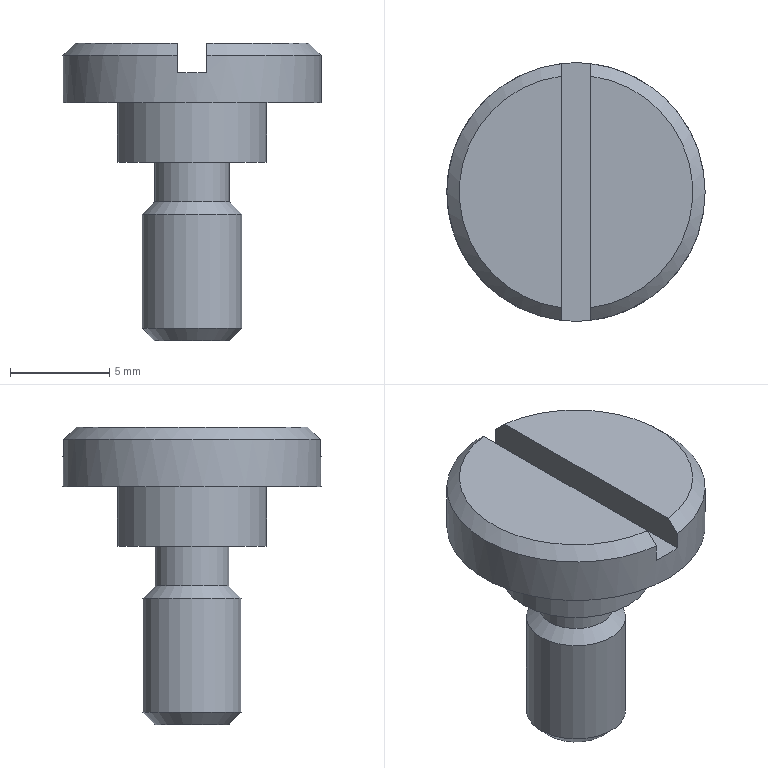Component | NX | DRILL_BUSHING_SCREW | 1 solid | 16 faces | box 13.01 x 13.01 x 15 mm | volume 650 mm3 | plane 8 | cone 4 | cylinder 4 | commonest cylinder face diameters 13.012 x1 7.512 x1 3.748 x1 5 x1
STEP:
#1=CARTESIAN_POINT('',(0.,0.,0.));
#2=DIRECTION('',(0.,0.,1.));
#3=DIRECTION('',(1.,0.,0.));
#4=AXIS2_PLACEMENT_3D('',#1,#2,#3);
#5=CARTESIAN_POINT('',(-1.25,94.806,-197.498));
#6=VERTEX_POINT('',#5);
#7=CARTESIAN_POINT('',(-1.25,106.47,-197.498));
#8=VERTEX_POINT('',#7);
#9=CARTESIAN_POINT('',(-1.25,86.638,-197.498));
#10=DIRECTION('',(0.,1.,0.));
#11=VECTOR('',#10,1.);
#12=LINE('',#9,#11);
#13=CARTESIAN_POINT('',(-2.,100.638,-197.498));
#14=DIRECTION('',(0.,0.,1.));
#15=DIRECTION('',(1.,0.,-0.));
#16=AXIS2_PLACEMENT_3D('',#13,#14,#15);
#17=PLANE('',#16);
#18=CARTESIAN_POINT('',(0.75,-14.));
#19=DIRECTION('',(0.,1.));
#20=VECTOR('',#19,1.);
#21=LINE('',#18,#20);
#22=(GEOMETRIC_REPRESENTATION_CONTEXT(2)PARAMETRIC_REPRESENTATION_CONTEXT()REPRESENTATION_CONTEXT('',''));
#23=DEFINITIONAL_REPRESENTATION('',(#21),#22);
#24=PCURVE('',#17,#23);
#25=CARTESIAN_POINT('',(-1.25,86.638,-198.998));
#26=DIRECTION('',(1.,0.,0.));
#27=DIRECTION('',(0.,0.,-1.));
#28=AXIS2_PLACEMENT_3D('',#25,#26,#27);
#29=PLANE('',#28);
#30=CARTESIAN_POINT('',(-1.5,0.));
#31=DIRECTION('',(0.,1.));
#32=VECTOR('',#31,1.);
#33=LINE('',#30,#32);
#34=(GEOMETRIC_REPRESENTATION_CONTEXT(2)PARAMETRIC_REPRESENTATION_CONTEXT()REPRESENTATION_CONTEXT('',''));
#35=DEFINITIONAL_REPRESENTATION('',(#33),#34);
#36=PCURVE('',#29,#35);
#37=SURFACE_CURVE('',#12,(#24,#36),.PCURVE_S1.);
#38=EDGE_CURVE('',#6,#8,#37,.T.);
#39=ORIENTED_EDGE('',*,*,#38,.F.);
#40=CARTESIAN_POINT('',(-2.,100.638,-197.498));
#41=DIRECTION('',(0.,0.,1.));
#42=DIRECTION('',(1.,0.,-0.));
#43=AXIS2_PLACEMENT_3D('',#40,#41,#42);
#44=CIRCLE('',#43,5.88);
#45=CARTESIAN_POINT('',(0.,0.));
#46=DIRECTION('',(1.,0.));
#47=AXIS2_PLACEMENT_2D('',#45,#46);
#48=CIRCLE('',#47,5.88);
#49=(GEOMETRIC_REPRESENTATION_CONTEXT(2)PARAMETRIC_REPRESENTATION_CONTEXT()REPRESENTATION_CONTEXT('',''));
#50=DEFINITIONAL_REPRESENTATION('',(#48),#49);
#51=PCURVE('',#17,#50);
#52=CARTESIAN_POINT('',(-2.,100.638,-198.12));
#53=DIRECTION('',(-0.,0.,-1.));
#54=DIRECTION('',(-1.,0.,0.));
#55=AXIS2_PLACEMENT_3D('',#52,#53,#54);
#56=CONICAL_SURFACE('',#55,6.506,0.7886);
#57=CARTESIAN_POINT('',(9.425,-0.622));
#58=DIRECTION('',(-1.,0.));
#59=VECTOR('',#58,1.);
#60=LINE('',#57,#59);
#61=(GEOMETRIC_REPRESENTATION_CONTEXT(2)PARAMETRIC_REPRESENTATION_CONTEXT()REPRESENTATION_CONTEXT('',''));
#62=DEFINITIONAL_REPRESENTATION('',(#60),#61);
#63=PCURVE('',#56,#62);
#64=SURFACE_CURVE('',#44,(#51,#63),.PCURVE_S1.);
#65=EDGE_CURVE('',#6,#8,#64,.T.);
#66=ORIENTED_EDGE('',*,*,#65,.T.);
#67=EDGE_LOOP('',(#39,#66));
#68=FACE_BOUND('',#67,.T.);
#69=ADVANCED_FACE('',(#68),#17,.T.);
#70=CARTESIAN_POINT('',(-1.25,94.176,-198.12));
#71=VERTEX_POINT('',#70);
#72=CARTESIAN_POINT('',(4.506,100.638,-198.12));
#73=VERTEX_POINT('',#72);
#74=CARTESIAN_POINT('',(-2.,100.638,-198.12));
#75=DIRECTION('',(0.,0.,1.));
#76=DIRECTION('',(1.,0.,-0.));
#77=AXIS2_PLACEMENT_3D('',#74,#75,#76);
#78=CIRCLE('',#77,6.506);
#79=CARTESIAN_POINT('',(9.425,-0.));
#80=DIRECTION('',(-1.,0.));
#81=VECTOR('',#80,1.);
#82=LINE('',#79,#81);
#83=(GEOMETRIC_REPRESENTATION_CONTEXT(2)PARAMETRIC_REPRESENTATION_CONTEXT()REPRESENTATION_CONTEXT('',''));
#84=DEFINITIONAL_REPRESENTATION('',(#82),#83);
#85=PCURVE('',#56,#84);
#86=CARTESIAN_POINT('',(-2.,100.638,-192.998));
#87=DIRECTION('',(0.,0.,1.));
#88=DIRECTION('',(1.,0.,-0.));
#89=AXIS2_PLACEMENT_3D('',#86,#87,#88);
#90=CYLINDRICAL_SURFACE('',#89,6.506);
#91=CARTESIAN_POINT('',(0.,-5.122));
#92=DIRECTION('',(1.,0.));
#93=VECTOR('',#92,1.);
#94=LINE('',#91,#93);
#95=(GEOMETRIC_REPRESENTATION_CONTEXT(2)PARAMETRIC_REPRESENTATION_CONTEXT()REPRESENTATION_CONTEXT('',''));
#96=DEFINITIONAL_REPRESENTATION('',(#94),#95);
#97=PCURVE('',#90,#96);
#98=SURFACE_CURVE('',#78,(#85,#97),.PCURVE_S1.);
#99=EDGE_CURVE('',#71,#73,#98,.T.);
#100=ORIENTED_EDGE('',*,*,#99,.T.);
#101=CARTESIAN_POINT('',(-1.25,107.101,-198.12));
#102=VERTEX_POINT('',#101);
#103=CARTESIAN_POINT('',(-2.,100.638,-198.12));
#104=DIRECTION('',(0.,0.,1.));
#105=DIRECTION('',(1.,0.,-0.));
#106=AXIS2_PLACEMENT_3D('',#103,#104,#105);
#107=CIRCLE('',#106,6.506);
#108=CARTESIAN_POINT('',(9.425,-0.));
#109=DIRECTION('',(-1.,0.));
#110=VECTOR('',#109,1.);
#111=LINE('',#108,#110);
#112=(GEOMETRIC_REPRESENTATION_CONTEXT(2)PARAMETRIC_REPRESENTATION_CONTEXT()REPRESENTATION_CONTEXT('',''));
#113=DEFINITIONAL_REPRESENTATION('',(#111),#112);
#114=PCURVE('',#56,#113);
#115=CARTESIAN_POINT('',(-6.283,-5.122));
#116=DIRECTION('',(1.,0.));
#117=VECTOR('',#116,1.);
#118=LINE('',#115,#117);
#119=(GEOMETRIC_REPRESENTATION_CONTEXT(2)PARAMETRIC_REPRESENTATION_CONTEXT()REPRESENTATION_CONTEXT('',''));
#120=DEFINITIONAL_REPRESENTATION('',(#118),#119);
#121=PCURVE('',#90,#120);
#122=SURFACE_CURVE('',#107,(#114,#121),.PCURVE_S1.);
#123=EDGE_CURVE('',#73,#102,#122,.T.);
#124=ORIENTED_EDGE('',*,*,#123,.T.);
#125=CARTESIAN_POINT('',(-1.25,107.101,-198.12));
#126=CARTESIAN_POINT('',(-1.25,106.891,-197.913));
#127=CARTESIAN_POINT('',(-1.25,106.681,-197.705));
#128=CARTESIAN_POINT('',(-1.25,106.47,-197.498));
#129=B_SPLINE_CURVE_WITH_KNOTS('',3,(#125,#126,#127,#128),.UNSPECIFIED.,.F.,.F.,(4,4),(0.,1.),.PIECEWISE_BEZIER_KNOTS.);
#130=CARTESIAN_POINT('',(1.686,-0.));
#131=CARTESIAN_POINT('',(1.699,-0.622));
#132=B_SPLINE_CURVE_WITH_KNOTS('',1,(#130,#131),.UNSPECIFIED.,.F.,.F.,(2,2),(0.,1.),.PIECEWISE_BEZIER_KNOTS.);
#133=(GEOMETRIC_REPRESENTATION_CONTEXT(2)PARAMETRIC_REPRESENTATION_CONTEXT()REPRESENTATION_CONTEXT('',''));
#134=DEFINITIONAL_REPRESENTATION('',(#132),#133);
#135=PCURVE('',#56,#134);
#136=CARTESIAN_POINT('',(-0.878,20.463));
#137=CARTESIAN_POINT('',(-1.085,20.252));
#138=CARTESIAN_POINT('',(-1.293,20.042));
#139=CARTESIAN_POINT('',(-1.5,19.832));
#140=B_SPLINE_CURVE_WITH_KNOTS('',3,(#136,#137,#138,#139),.UNSPECIFIED.,.F.,.F.,(4,4),(0.,1.),.PIECEWISE_BEZIER_KNOTS.);
#141=(GEOMETRIC_REPRESENTATION_CONTEXT(2)PARAMETRIC_REPRESENTATION_CONTEXT()REPRESENTATION_CONTEXT('',''));
#142=DEFINITIONAL_REPRESENTATION('',(#140),#141);
#143=PCURVE('',#29,#142);
#144=SURFACE_CURVE('',#129,(#135,#143),.PCURVE_S1.);
#145=EDGE_CURVE('',#102,#8,#144,.T.);
#146=ORIENTED_EDGE('',*,*,#145,.T.);
#147=ORIENTED_EDGE('',*,*,#65,.F.);
#148=CARTESIAN_POINT('',(-1.25,94.806,-197.498));
#149=CARTESIAN_POINT('',(-1.25,94.596,-197.705));
#150=CARTESIAN_POINT('',(-1.25,94.386,-197.913));
#151=CARTESIAN_POINT('',(-1.25,94.176,-198.12));
#152=B_SPLINE_CURVE_WITH_KNOTS('',3,(#148,#149,#150,#151),.UNSPECIFIED.,.F.,.F.,(4,4),(0.,1.),.PIECEWISE_BEZIER_KNOTS.);
#153=CARTESIAN_POINT('',(4.584,-0.622));
#154=CARTESIAN_POINT('',(4.597,0.));
#155=B_SPLINE_CURVE_WITH_KNOTS('',1,(#153,#154),.UNSPECIFIED.,.F.,.F.,(2,2),(0.,1.),.PIECEWISE_BEZIER_KNOTS.);
#156=(GEOMETRIC_REPRESENTATION_CONTEXT(2)PARAMETRIC_REPRESENTATION_CONTEXT()REPRESENTATION_CONTEXT('',''));
#157=DEFINITIONAL_REPRESENTATION('',(#155),#156);
#158=PCURVE('',#56,#157);
#159=CARTESIAN_POINT('',(-1.5,8.168));
#160=CARTESIAN_POINT('',(-1.293,7.958));
#161=CARTESIAN_POINT('',(-1.085,7.748));
#162=CARTESIAN_POINT('',(-0.878,7.537));
#163=B_SPLINE_CURVE_WITH_KNOTS('',3,(#159,#160,#161,#162),.UNSPECIFIED.,.F.,.F.,(4,4),(0.,1.),.PIECEWISE_BEZIER_KNOTS.);
#164=(GEOMETRIC_REPRESENTATION_CONTEXT(2)PARAMETRIC_REPRESENTATION_CONTEXT()REPRESENTATION_CONTEXT('',''));
#165=DEFINITIONAL_REPRESENTATION('',(#163),#164);
#166=PCURVE('',#29,#165);
#167=SURFACE_CURVE('',#152,(#158,#166),.PCURVE_S1.);
#168=EDGE_CURVE('',#6,#71,#167,.T.);
#169=ORIENTED_EDGE('',*,*,#168,.T.);
#170=EDGE_LOOP('',(#100,#124,#146,#147,#169));
#171=FACE_BOUND('',#170,.T.);
#172=ADVANCED_FACE('',(#171),#56,.T.);
#173=CARTESIAN_POINT('',(-0.122,100.638,-212.498));
#174=VERTEX_POINT('',#173);
#175=CARTESIAN_POINT('',(-2.,100.638,-212.498));
#176=DIRECTION('',(0.,0.,1.));
#177=DIRECTION('',(1.,0.,-0.));
#178=AXIS2_PLACEMENT_3D('',#175,#176,#177);
#179=CIRCLE('',#178,1.878);
#180=CARTESIAN_POINT('',(-2.,100.638,-212.498));
#181=DIRECTION('',(0.,0.,1.));
#182=DIRECTION('',(1.,0.,-0.));
#183=AXIS2_PLACEMENT_3D('',#180,#181,#182);
#184=PLANE('',#183);
#185=CARTESIAN_POINT('',(0.,0.));
#186=DIRECTION('',(1.,0.));
#187=AXIS2_PLACEMENT_2D('',#185,#186);
#188=CIRCLE('',#187,1.878);
#189=(GEOMETRIC_REPRESENTATION_CONTEXT(2)PARAMETRIC_REPRESENTATION_CONTEXT()REPRESENTATION_CONTEXT('',''));
#190=DEFINITIONAL_REPRESENTATION('',(#188),#189);
#191=PCURVE('',#184,#190);
#192=CARTESIAN_POINT('',(-2.,100.638,-212.498));
#193=DIRECTION('',(0.,0.,1.));
#194=DIRECTION('',(1.,0.,-0.));
#195=AXIS2_PLACEMENT_3D('',#192,#193,#194);
#196=CONICAL_SURFACE('',#195,1.878,0.7822);
#197=CARTESIAN_POINT('',(0.,0.));
#198=DIRECTION('',(1.,0.));
#199=VECTOR('',#198,1.);
#200=LINE('',#197,#199);
#201=(GEOMETRIC_REPRESENTATION_CONTEXT(2)PARAMETRIC_REPRESENTATION_CONTEXT()REPRESENTATION_CONTEXT('',''));
#202=DEFINITIONAL_REPRESENTATION('',(#200),#201);
#203=PCURVE('',#196,#202);
#204=SURFACE_CURVE('',#179,(#191,#203),.PCURVE_S1.);
#205=EDGE_CURVE('',#174,#174,#204,.T.);
#206=ORIENTED_EDGE('',*,*,#205,.F.);
#207=EDGE_LOOP('',(#206));
#208=FACE_BOUND('',#207,.T.);
#209=ADVANCED_FACE('',(#208),#184,.F.);
#210=CARTESIAN_POINT('',(-2.75,106.47,-197.498));
#211=VERTEX_POINT('',#210);
#212=CARTESIAN_POINT('',(-2.75,94.806,-197.498));
#213=VERTEX_POINT('',#212);
#214=CARTESIAN_POINT('',(-2.75,114.638,-197.498));
#215=DIRECTION('',(0.,-1.,0.));
#216=VECTOR('',#215,1.);
#217=LINE('',#214,#216);
#218=CARTESIAN_POINT('',(-2.,100.638,-197.498));
#219=DIRECTION('',(0.,0.,1.));
#220=DIRECTION('',(1.,0.,-0.));
#221=AXIS2_PLACEMENT_3D('',#218,#219,#220);
#222=PLANE('',#221);
#223=CARTESIAN_POINT('',(-0.75,14.));
#224=DIRECTION('',(0.,-1.));
#225=VECTOR('',#224,1.);
#226=LINE('',#223,#225);
#227=(GEOMETRIC_REPRESENTATION_CONTEXT(2)PARAMETRIC_REPRESENTATION_CONTEXT()REPRESENTATION_CONTEXT('',''));
#228=DEFINITIONAL_REPRESENTATION('',(#226),#227);
#229=PCURVE('',#222,#228);
#230=CARTESIAN_POINT('',(-2.75,114.638,-198.998));
#231=DIRECTION('',(-1.,0.,0.));
#232=DIRECTION('',(0.,0.,1.));
#233=AXIS2_PLACEMENT_3D('',#230,#231,#232);
#234=PLANE('',#233);
#235=CARTESIAN_POINT('',(1.5,0.));
#236=DIRECTION('',(0.,-1.));
#237=VECTOR('',#236,1.);
#238=LINE('',#235,#237);
#239=(GEOMETRIC_REPRESENTATION_CONTEXT(2)PARAMETRIC_REPRESENTATION_CONTEXT()REPRESENTATION_CONTEXT('',''));
#240=DEFINITIONAL_REPRESENTATION('',(#238),#239);
#241=PCURVE('',#234,#240);
#242=SURFACE_CURVE('',#217,(#229,#241),.PCURVE_S1.);
#243=EDGE_CURVE('',#211,#213,#242,.T.);
#244=ORIENTED_EDGE('',*,*,#243,.F.);
#245=CARTESIAN_POINT('',(-2.,100.638,-197.498));
#246=DIRECTION('',(0.,0.,1.));
#247=DIRECTION('',(1.,0.,-0.));
#248=AXIS2_PLACEMENT_3D('',#245,#246,#247);
#249=CIRCLE('',#248,5.88);
#250=CARTESIAN_POINT('',(0.,0.));
#251=DIRECTION('',(1.,0.));
#252=AXIS2_PLACEMENT_2D('',#250,#251);
#253=CIRCLE('',#252,5.88);
#254=(GEOMETRIC_REPRESENTATION_CONTEXT(2)PARAMETRIC_REPRESENTATION_CONTEXT()REPRESENTATION_CONTEXT('',''));
#255=DEFINITIONAL_REPRESENTATION('',(#253),#254);
#256=PCURVE('',#222,#255);
#257=CARTESIAN_POINT('',(-2.,100.638,-198.12));
#258=DIRECTION('',(-0.,0.,-1.));
#259=DIRECTION('',(-1.,0.,0.));
#260=AXIS2_PLACEMENT_3D('',#257,#258,#259);
#261=CONICAL_SURFACE('',#260,6.506,0.7886);
#262=CARTESIAN_POINT('',(9.425,-0.622));
#263=DIRECTION('',(-1.,-0.));
#264=VECTOR('',#263,1.);
#265=LINE('',#262,#264);
#266=(GEOMETRIC_REPRESENTATION_CONTEXT(2)PARAMETRIC_REPRESENTATION_CONTEXT()REPRESENTATION_CONTEXT('',''));
#267=DEFINITIONAL_REPRESENTATION('',(#265),#266);
#268=PCURVE('',#261,#267);
#269=SURFACE_CURVE('',#249,(#256,#268),.PCURVE_S1.);
#270=EDGE_CURVE('',#211,#213,#269,.T.);
#271=ORIENTED_EDGE('',*,*,#270,.T.);
#272=EDGE_LOOP('',(#244,#271));
#273=FACE_BOUND('',#272,.T.);
#274=ADVANCED_FACE('',(#273),#222,.T.);
#275=CARTESIAN_POINT('',(-2.75,107.101,-198.12));
#276=VERTEX_POINT('',#275);
#277=CARTESIAN_POINT('',(-2.75,94.176,-198.12));
#278=VERTEX_POINT('',#277);
#279=CARTESIAN_POINT('',(-2.,100.638,-198.12));
#280=DIRECTION('',(0.,0.,1.));
#281=DIRECTION('',(1.,0.,-0.));
#282=AXIS2_PLACEMENT_3D('',#279,#280,#281);
#283=CIRCLE('',#282,6.506);
#284=CARTESIAN_POINT('',(9.425,-0.));
#285=DIRECTION('',(-1.,-0.));
#286=VECTOR('',#285,1.);
#287=LINE('',#284,#286);
#288=(GEOMETRIC_REPRESENTATION_CONTEXT(2)PARAMETRIC_REPRESENTATION_CONTEXT()REPRESENTATION_CONTEXT('',''));
#289=DEFINITIONAL_REPRESENTATION('',(#287),#288);
#290=PCURVE('',#261,#289);
#291=CARTESIAN_POINT('',(0.,-5.122));
#292=DIRECTION('',(1.,0.));
#293=VECTOR('',#292,1.);
#294=LINE('',#291,#293);
#295=(GEOMETRIC_REPRESENTATION_CONTEXT(2)PARAMETRIC_REPRESENTATION_CONTEXT()REPRESENTATION_CONTEXT('',''));
#296=DEFINITIONAL_REPRESENTATION('',(#294),#295);
#297=PCURVE('',#90,#296);
#298=SURFACE_CURVE('',#283,(#290,#297),.PCURVE_S1.);
#299=EDGE_CURVE('',#276,#278,#298,.T.);
#300=ORIENTED_EDGE('',*,*,#299,.T.);
#301=CARTESIAN_POINT('',(-2.75,94.176,-198.12));
#302=CARTESIAN_POINT('',(-2.75,94.386,-197.913));
#303=CARTESIAN_POINT('',(-2.75,94.596,-197.705));
#304=CARTESIAN_POINT('',(-2.75,94.806,-197.498));
#305=B_SPLINE_CURVE_WITH_KNOTS('',3,(#301,#302,#303,#304),.UNSPECIFIED.,.F.,.F.,(4,4),(0.,1.),.PIECEWISE_BEZIER_KNOTS.);
#306=CARTESIAN_POINT('',(4.828,0.));
#307=CARTESIAN_POINT('',(4.84,-0.622));
#308=B_SPLINE_CURVE_WITH_KNOTS('',1,(#306,#307),.UNSPECIFIED.,.F.,.F.,(2,2),(0.,1.),.PIECEWISE_BEZIER_KNOTS.);
#309=(GEOMETRIC_REPRESENTATION_CONTEXT(2)PARAMETRIC_REPRESENTATION_CONTEXT()REPRESENTATION_CONTEXT('',''));
#310=DEFINITIONAL_REPRESENTATION('',(#308),#309);
#311=PCURVE('',#261,#310);
#312=CARTESIAN_POINT('',(0.878,-20.463));
#313=CARTESIAN_POINT('',(1.085,-20.252));
#314=CARTESIAN_POINT('',(1.293,-20.042));
#315=CARTESIAN_POINT('',(1.5,-19.832));
#316=B_SPLINE_CURVE_WITH_KNOTS('',3,(#312,#313,#314,#315),.UNSPECIFIED.,.F.,.F.,(4,4),(0.,1.),.PIECEWISE_BEZIER_KNOTS.);
#317=(GEOMETRIC_REPRESENTATION_CONTEXT(2)PARAMETRIC_REPRESENTATION_CONTEXT()REPRESENTATION_CONTEXT('',''));
#318=DEFINITIONAL_REPRESENTATION('',(#316),#317);
#319=PCURVE('',#234,#318);
#320=SURFACE_CURVE('',#305,(#311,#319),.PCURVE_S1.);
#321=EDGE_CURVE('',#278,#213,#320,.T.);
#322=ORIENTED_EDGE('',*,*,#321,.T.);
#323=ORIENTED_EDGE('',*,*,#270,.F.);
#324=CARTESIAN_POINT('',(-2.75,106.47,-197.498));
#325=CARTESIAN_POINT('',(-2.75,106.681,-197.705));
#326=CARTESIAN_POINT('',(-2.75,106.891,-197.913));
#327=CARTESIAN_POINT('',(-2.75,107.101,-198.12));
#328=B_SPLINE_CURVE_WITH_KNOTS('',3,(#324,#325,#326,#327),.UNSPECIFIED.,.F.,.F.,(4,4),(0.,1.),.PIECEWISE_BEZIER_KNOTS.);
#329=CARTESIAN_POINT('',(7.726,-0.622));
#330=CARTESIAN_POINT('',(7.738,-0.));
#331=B_SPLINE_CURVE_WITH_KNOTS('',1,(#329,#330),.UNSPECIFIED.,.F.,.F.,(2,2),(0.,1.),.PIECEWISE_BEZIER_KNOTS.);
#332=(GEOMETRIC_REPRESENTATION_CONTEXT(2)PARAMETRIC_REPRESENTATION_CONTEXT()REPRESENTATION_CONTEXT('',''));
#333=DEFINITIONAL_REPRESENTATION('',(#331),#332);
#334=PCURVE('',#261,#333);
#335=CARTESIAN_POINT('',(1.5,-8.168));
#336=CARTESIAN_POINT('',(1.293,-7.958));
#337=CARTESIAN_POINT('',(1.085,-7.748));
#338=CARTESIAN_POINT('',(0.878,-7.537));
#339=B_SPLINE_CURVE_WITH_KNOTS('',3,(#335,#336,#337,#338),.UNSPECIFIED.,.F.,.F.,(4,4),(0.,1.),.PIECEWISE_BEZIER_KNOTS.);
#340=(GEOMETRIC_REPRESENTATION_CONTEXT(2)PARAMETRIC_REPRESENTATION_CONTEXT()REPRESENTATION_CONTEXT('',''));
#341=DEFINITIONAL_REPRESENTATION('',(#339),#340);
#342=PCURVE('',#234,#341);
#343=SURFACE_CURVE('',#328,(#334,#342),.PCURVE_S1.);
#344=EDGE_CURVE('',#211,#276,#343,.T.);
#345=ORIENTED_EDGE('',*,*,#344,.T.);
#346=EDGE_LOOP('',(#300,#322,#323,#345));
#347=FACE_BOUND('',#346,.T.);
#348=ADVANCED_FACE('',(#347),#261,.T.);
#349=ORIENTED_EDGE('',*,*,#123,.F.);
#350=CARTESIAN_POINT('',(4.506,100.638,-200.5));
#351=VERTEX_POINT('',#350);
#352=CARTESIAN_POINT('',(4.506,100.638,-200.5));
#353=CARTESIAN_POINT('',(4.506,100.638,-198.12));
#354=B_SPLINE_CURVE_WITH_KNOTS('',1,(#352,#353),.UNSPECIFIED.,.F.,.F.,(2,2),(-7.502,-5.122),.PIECEWISE_BEZIER_KNOTS.);
#355=CARTESIAN_POINT('',(0.,0.));
#356=DIRECTION('',(0.,1.));
#357=VECTOR('',#356,1.);
#358=LINE('',#355,#357);
#359=(GEOMETRIC_REPRESENTATION_CONTEXT(2)PARAMETRIC_REPRESENTATION_CONTEXT()REPRESENTATION_CONTEXT('',''));
#360=DEFINITIONAL_REPRESENTATION('',(#358),#359);
#361=PCURVE('',#90,#360);
#362=CARTESIAN_POINT('',(6.283,0.));
#363=DIRECTION('',(0.,1.));
#364=VECTOR('',#363,1.);
#365=LINE('',#362,#364);
#366=(GEOMETRIC_REPRESENTATION_CONTEXT(2)PARAMETRIC_REPRESENTATION_CONTEXT()REPRESENTATION_CONTEXT('',''));
#367=DEFINITIONAL_REPRESENTATION('',(#365),#366);
#368=PCURVE('',#90,#367);
#369=SEAM_CURVE('',#354,(#361,#368),.PCURVE_S1.);
#370=EDGE_CURVE('',#351,#73,#369,.T.);
#371=ORIENTED_EDGE('',*,*,#370,.F.);
#372=CARTESIAN_POINT('',(-2.,100.638,-200.5));
#373=DIRECTION('',(0.,0.,1.));
#374=DIRECTION('',(1.,0.,-0.));
#375=AXIS2_PLACEMENT_3D('',#372,#373,#374);
#376=CIRCLE('',#375,6.506);
#377=CARTESIAN_POINT('',(0.,-7.502));
#378=DIRECTION('',(1.,0.));
#379=VECTOR('',#378,1.);
#380=LINE('',#377,#379);
#381=(GEOMETRIC_REPRESENTATION_CONTEXT(2)PARAMETRIC_REPRESENTATION_CONTEXT()REPRESENTATION_CONTEXT('',''));
#382=DEFINITIONAL_REPRESENTATION('',(#380),#381);
#383=PCURVE('',#90,#382);
#384=CARTESIAN_POINT('',(1.756,100.638,-200.5));
#385=DIRECTION('',(0.,0.,1.));
#386=DIRECTION('',(1.,0.,-0.));
#387=AXIS2_PLACEMENT_3D('',#384,#385,#386);
#388=PLANE('',#387);
#389=CARTESIAN_POINT('',(-3.756,0.));
#390=DIRECTION('',(1.,0.));
#391=AXIS2_PLACEMENT_2D('',#389,#390);
#392=CIRCLE('',#391,6.506);
#393=(GEOMETRIC_REPRESENTATION_CONTEXT(2)PARAMETRIC_REPRESENTATION_CONTEXT()REPRESENTATION_CONTEXT('',''));
#394=DEFINITIONAL_REPRESENTATION('',(#392),#393);
#395=PCURVE('',#388,#394);
#396=SURFACE_CURVE('',#376,(#383,#395),.PCURVE_S1.);
#397=EDGE_CURVE('',#351,#351,#396,.T.);
#398=ORIENTED_EDGE('',*,*,#397,.T.);
#399=ORIENTED_EDGE('',*,*,#370,.T.);
#400=ORIENTED_EDGE('',*,*,#99,.F.);
#401=CARTESIAN_POINT('',(-1.25,94.176,-198.998));
#402=VERTEX_POINT('',#401);
#403=CARTESIAN_POINT('',(-1.25,94.176,-192.998));
#404=DIRECTION('',(-0.,0.,-1.));
#405=VECTOR('',#404,1.);
#406=LINE('',#403,#405);
#407=CARTESIAN_POINT('',(4.828,0.));
#408=DIRECTION('',(0.,-1.));
#409=VECTOR('',#408,1.);
#410=LINE('',#407,#409);
#411=(GEOMETRIC_REPRESENTATION_CONTEXT(2)PARAMETRIC_REPRESENTATION_CONTEXT()REPRESENTATION_CONTEXT('',''));
#412=DEFINITIONAL_REPRESENTATION('',(#410),#411);
#413=PCURVE('',#90,#412);
#414=CARTESIAN_POINT('',(-6.,7.537));
#415=DIRECTION('',(1.,0.));
#416=VECTOR('',#415,1.);
#417=LINE('',#414,#416);
#418=(GEOMETRIC_REPRESENTATION_CONTEXT(2)PARAMETRIC_REPRESENTATION_CONTEXT()REPRESENTATION_CONTEXT('',''));
#419=DEFINITIONAL_REPRESENTATION('',(#417),#418);
#420=PCURVE('',#29,#419);
#421=SURFACE_CURVE('',#406,(#413,#420),.PCURVE_S1.);
#422=EDGE_CURVE('',#71,#402,#421,.T.);
#423=ORIENTED_EDGE('',*,*,#422,.T.);
#424=CARTESIAN_POINT('',(-2.75,94.176,-198.998));
#425=VERTEX_POINT('',#424);
#426=CARTESIAN_POINT('',(-2.,100.638,-198.998));
#427=DIRECTION('',(0.,0.,1.));
#428=DIRECTION('',(0.,1.,0.));
#429=AXIS2_PLACEMENT_3D('',#426,#427,#428);
#430=CIRCLE('',#429,6.506);
#431=CARTESIAN_POINT('',(1.571,-6.));
#432=DIRECTION('',(1.,0.));
#433=VECTOR('',#432,1.);
#434=LINE('',#431,#433);
#435=(GEOMETRIC_REPRESENTATION_CONTEXT(2)PARAMETRIC_REPRESENTATION_CONTEXT()REPRESENTATION_CONTEXT('',''));
#436=DEFINITIONAL_REPRESENTATION('',(#434),#435);
#437=PCURVE('',#90,#436);
#438=CARTESIAN_POINT('',(-2.,100.638,-198.998));
#439=DIRECTION('',(0.,0.,1.));
#440=DIRECTION('',(0.,1.,0.));
#441=AXIS2_PLACEMENT_3D('',#438,#439,#440);
#442=PLANE('',#441);
#443=CARTESIAN_POINT('',(0.,0.));
#444=DIRECTION('',(1.,0.));
#445=AXIS2_PLACEMENT_2D('',#443,#444);
#446=CIRCLE('',#445,6.506);
#447=(GEOMETRIC_REPRESENTATION_CONTEXT(2)PARAMETRIC_REPRESENTATION_CONTEXT()REPRESENTATION_CONTEXT('',''));
#448=DEFINITIONAL_REPRESENTATION('',(#446),#447);
#449=PCURVE('',#442,#448);
#450=SURFACE_CURVE('',#430,(#437,#449),.PCURVE_S1.);
#451=EDGE_CURVE('',#425,#402,#450,.T.);
#452=ORIENTED_EDGE('',*,*,#451,.F.);
#453=CARTESIAN_POINT('',(-2.75,94.176,-192.998));
#454=DIRECTION('',(0.,0.,1.));
#455=VECTOR('',#454,1.);
#456=LINE('',#453,#455);
#457=CARTESIAN_POINT('',(4.597,0.));
#458=DIRECTION('',(0.,1.));
#459=VECTOR('',#458,1.);
#460=LINE('',#457,#459);
#461=(GEOMETRIC_REPRESENTATION_CONTEXT(2)PARAMETRIC_REPRESENTATION_CONTEXT()REPRESENTATION_CONTEXT('',''));
#462=DEFINITIONAL_REPRESENTATION('',(#460),#461);
#463=PCURVE('',#90,#462);
#464=CARTESIAN_POINT('',(6.,-20.463));
#465=DIRECTION('',(1.,0.));
#466=VECTOR('',#465,1.);
#467=LINE('',#464,#466);
#468=(GEOMETRIC_REPRESENTATION_CONTEXT(2)PARAMETRIC_REPRESENTATION_CONTEXT()REPRESENTATION_CONTEXT('',''));
#469=DEFINITIONAL_REPRESENTATION('',(#467),#468);
#470=PCURVE('',#234,#469);
#471=SURFACE_CURVE('',#456,(#463,#470),.PCURVE_S1.);
#472=EDGE_CURVE('',#425,#278,#471,.T.);
#473=ORIENTED_EDGE('',*,*,#472,.T.);
#474=ORIENTED_EDGE('',*,*,#299,.F.);
#475=CARTESIAN_POINT('',(-2.75,107.101,-198.998));
#476=VERTEX_POINT('',#475);
#477=CARTESIAN_POINT('',(-2.75,107.101,-192.998));
#478=DIRECTION('',(-0.,0.,-1.));
#479=VECTOR('',#478,1.);
#480=LINE('',#477,#479);
#481=CARTESIAN_POINT('',(1.686,0.));
#482=DIRECTION('',(0.,-1.));
#483=VECTOR('',#482,1.);
#484=LINE('',#481,#483);
#485=(GEOMETRIC_REPRESENTATION_CONTEXT(2)PARAMETRIC_REPRESENTATION_CONTEXT()REPRESENTATION_CONTEXT('',''));
#486=DEFINITIONAL_REPRESENTATION('',(#484),#485);
#487=PCURVE('',#90,#486);
#488=CARTESIAN_POINT('',(6.,-7.537));
#489=DIRECTION('',(-1.,0.));
#490=VECTOR('',#489,1.);
#491=LINE('',#488,#490);
#492=(GEOMETRIC_REPRESENTATION_CONTEXT(2)PARAMETRIC_REPRESENTATION_CONTEXT()REPRESENTATION_CONTEXT('',''));
#493=DEFINITIONAL_REPRESENTATION('',(#491),#492);
#494=PCURVE('',#234,#493);
#495=SURFACE_CURVE('',#480,(#487,#494),.PCURVE_S1.);
#496=EDGE_CURVE('',#276,#476,#495,.T.);
#497=ORIENTED_EDGE('',*,*,#496,.T.);
#498=CARTESIAN_POINT('',(-1.25,107.101,-198.998));
#499=VERTEX_POINT('',#498);
#500=CARTESIAN_POINT('',(-2.,100.638,-198.998));
#501=DIRECTION('',(0.,0.,1.));
#502=DIRECTION('',(0.,1.,0.));
#503=AXIS2_PLACEMENT_3D('',#500,#501,#502);
#504=CIRCLE('',#503,6.506);
#505=CARTESIAN_POINT('',(-4.712,-6.));
#506=DIRECTION('',(1.,0.));
#507=VECTOR('',#506,1.);
#508=LINE('',#505,#507);
#509=(GEOMETRIC_REPRESENTATION_CONTEXT(2)PARAMETRIC_REPRESENTATION_CONTEXT()REPRESENTATION_CONTEXT('',''));
#510=DEFINITIONAL_REPRESENTATION('',(#508),#509);
#511=PCURVE('',#90,#510);
#512=CARTESIAN_POINT('',(0.,0.));
#513=DIRECTION('',(1.,0.));
#514=AXIS2_PLACEMENT_2D('',#512,#513);
#515=CIRCLE('',#514,6.506);
#516=(GEOMETRIC_REPRESENTATION_CONTEXT(2)PARAMETRIC_REPRESENTATION_CONTEXT()REPRESENTATION_CONTEXT('',''));
#517=DEFINITIONAL_REPRESENTATION('',(#515),#516);
#518=PCURVE('',#442,#517);
#519=SURFACE_CURVE('',#504,(#511,#518),.PCURVE_S1.);
#520=EDGE_CURVE('',#499,#476,#519,.T.);
#521=ORIENTED_EDGE('',*,*,#520,.F.);
#522=CARTESIAN_POINT('',(-1.25,107.101,-192.998));
#523=DIRECTION('',(0.,0.,1.));
#524=VECTOR('',#523,1.);
#525=LINE('',#522,#524);
#526=CARTESIAN_POINT('',(1.455,0.));
#527=DIRECTION('',(0.,1.));
#528=VECTOR('',#527,1.);
#529=LINE('',#526,#528);
#530=(GEOMETRIC_REPRESENTATION_CONTEXT(2)PARAMETRIC_REPRESENTATION_CONTEXT()REPRESENTATION_CONTEXT('',''));
#531=DEFINITIONAL_REPRESENTATION('',(#529),#530);
#532=PCURVE('',#90,#531);
#533=CARTESIAN_POINT('',(-6.,20.463));
#534=DIRECTION('',(-1.,0.));
#535=VECTOR('',#534,1.);
#536=LINE('',#533,#535);
#537=(GEOMETRIC_REPRESENTATION_CONTEXT(2)PARAMETRIC_REPRESENTATION_CONTEXT()REPRESENTATION_CONTEXT('',''));
#538=DEFINITIONAL_REPRESENTATION('',(#536),#537);
#539=PCURVE('',#29,#538);
#540=SURFACE_CURVE('',#525,(#532,#539),.PCURVE_S1.);
#541=EDGE_CURVE('',#499,#102,#540,.T.);
#542=ORIENTED_EDGE('',*,*,#541,.T.);
#543=EDGE_LOOP('',(#349,#371,#398,#399,#400,#423,#452,#473,#474,#497,#521,#542));
#544=FACE_BOUND('',#543,.T.);
#545=ADVANCED_FACE('',(#544),#90,.T.);
#546=ORIENTED_EDGE('',*,*,#397,.F.);
#547=EDGE_LOOP('',(#546));
#548=FACE_BOUND('',#547,.T.);
#549=CARTESIAN_POINT('',(1.756,100.638,-200.5));
#550=VERTEX_POINT('',#549);
#551=CARTESIAN_POINT('',(-2.,100.638,-200.5));
#552=DIRECTION('',(0.,0.,1.));
#553=DIRECTION('',(1.,0.,-0.));
#554=AXIS2_PLACEMENT_3D('',#551,#552,#553);
#555=CIRCLE('',#554,3.756);
#556=CARTESIAN_POINT('',(-3.756,0.));
#557=DIRECTION('',(1.,0.));
#558=AXIS2_PLACEMENT_2D('',#556,#557);
#559=CIRCLE('',#558,3.756);
#560=(GEOMETRIC_REPRESENTATION_CONTEXT(2)PARAMETRIC_REPRESENTATION_CONTEXT()REPRESENTATION_CONTEXT('',''));
#561=DEFINITIONAL_REPRESENTATION('',(#559),#560);
#562=PCURVE('',#388,#561);
#563=CARTESIAN_POINT('',(-2.,100.638,-192.998));
#564=DIRECTION('',(0.,0.,1.));
#565=DIRECTION('',(1.,0.,-0.));
#566=AXIS2_PLACEMENT_3D('',#563,#564,#565);
#567=CYLINDRICAL_SURFACE('',#566,3.756);
#568=CARTESIAN_POINT('',(0.,-7.502));
#569=DIRECTION('',(1.,0.));
#570=VECTOR('',#569,1.);
#571=LINE('',#568,#570);
#572=(GEOMETRIC_REPRESENTATION_CONTEXT(2)PARAMETRIC_REPRESENTATION_CONTEXT()REPRESENTATION_CONTEXT('',''));
#573=DEFINITIONAL_REPRESENTATION('',(#571),#572);
#574=PCURVE('',#567,#573);
#575=SURFACE_CURVE('',#555,(#562,#574),.PCURVE_S1.);
#576=EDGE_CURVE('',#550,#550,#575,.T.);
#577=ORIENTED_EDGE('',*,*,#576,.T.);
#578=EDGE_LOOP('',(#577));
#579=FACE_BOUND('',#578,.T.);
#580=ADVANCED_FACE('',(#548,#579),#388,.F.);
#581=ORIENTED_EDGE('',*,*,#576,.F.);
#582=CARTESIAN_POINT('',(1.756,100.638,-203.5));
#583=VERTEX_POINT('',#582);
#584=CARTESIAN_POINT('',(1.756,100.638,-203.5));
#585=CARTESIAN_POINT('',(1.756,100.638,-200.5));
#586=B_SPLINE_CURVE_WITH_KNOTS('',1,(#584,#585),.UNSPECIFIED.,.F.,.F.,(2,2),(-10.502,-7.502),.PIECEWISE_BEZIER_KNOTS.);
#587=CARTESIAN_POINT('',(0.,0.));
#588=DIRECTION('',(0.,1.));
#589=VECTOR('',#588,1.);
#590=LINE('',#587,#589);
#591=(GEOMETRIC_REPRESENTATION_CONTEXT(2)PARAMETRIC_REPRESENTATION_CONTEXT()REPRESENTATION_CONTEXT('',''));
#592=DEFINITIONAL_REPRESENTATION('',(#590),#591);
#593=PCURVE('',#567,#592);
#594=CARTESIAN_POINT('',(6.283,0.));
#595=DIRECTION('',(0.,1.));
#596=VECTOR('',#595,1.);
#597=LINE('',#594,#596);
#598=(GEOMETRIC_REPRESENTATION_CONTEXT(2)PARAMETRIC_REPRESENTATION_CONTEXT()REPRESENTATION_CONTEXT('',''));
#599=DEFINITIONAL_REPRESENTATION('',(#597),#598);
#600=PCURVE('',#567,#599);
#601=SEAM_CURVE('',#586,(#593,#600),.PCURVE_S1.);
#602=EDGE_CURVE('',#583,#550,#601,.T.);
#603=ORIENTED_EDGE('',*,*,#602,.F.);
#604=CARTESIAN_POINT('',(-2.,100.638,-203.5));
#605=DIRECTION('',(0.,0.,1.));
#606=DIRECTION('',(1.,0.,-0.));
#607=AXIS2_PLACEMENT_3D('',#604,#605,#606);
#608=CIRCLE('',#607,3.756);
#609=CARTESIAN_POINT('',(0.,-10.502));
#610=DIRECTION('',(1.,0.));
#611=VECTOR('',#610,1.);
#612=LINE('',#609,#611);
#613=(GEOMETRIC_REPRESENTATION_CONTEXT(2)PARAMETRIC_REPRESENTATION_CONTEXT()REPRESENTATION_CONTEXT('',''));
#614=DEFINITIONAL_REPRESENTATION('',(#612),#613);
#615=PCURVE('',#567,#614);
#616=CARTESIAN_POINT('',(-0.126,100.638,-203.5));
#617=DIRECTION('',(0.,0.,1.));
#618=DIRECTION('',(1.,0.,-0.));
#619=AXIS2_PLACEMENT_3D('',#616,#617,#618);
#620=PLANE('',#619);
#621=CARTESIAN_POINT('',(-1.874,0.));
#622=DIRECTION('',(1.,0.));
#623=AXIS2_PLACEMENT_2D('',#621,#622);
#624=CIRCLE('',#623,3.756);
#625=(GEOMETRIC_REPRESENTATION_CONTEXT(2)PARAMETRIC_REPRESENTATION_CONTEXT()REPRESENTATION_CONTEXT('',''));
#626=DEFINITIONAL_REPRESENTATION('',(#624),#625);
#627=PCURVE('',#620,#626);
#628=SURFACE_CURVE('',#608,(#615,#627),.PCURVE_S1.);
#629=EDGE_CURVE('',#583,#583,#628,.T.);
#630=ORIENTED_EDGE('',*,*,#629,.T.);
#631=ORIENTED_EDGE('',*,*,#602,.T.);
#632=EDGE_LOOP('',(#581,#603,#630,#631));
#633=FACE_BOUND('',#632,.T.);
#634=ADVANCED_FACE('',(#633),#567,.T.);
#635=ORIENTED_EDGE('',*,*,#629,.F.);
#636=EDGE_LOOP('',(#635));
#637=FACE_BOUND('',#636,.T.);
#638=CARTESIAN_POINT('',(-0.126,100.638,-203.5));
#639=VERTEX_POINT('',#638);
#640=CARTESIAN_POINT('',(-2.,100.638,-203.5));
#641=DIRECTION('',(0.,0.,1.));
#642=DIRECTION('',(1.,0.,-0.));
#643=AXIS2_PLACEMENT_3D('',#640,#641,#642);
#644=CIRCLE('',#643,1.874);
#645=CARTESIAN_POINT('',(-1.874,0.));
#646=DIRECTION('',(1.,0.));
#647=AXIS2_PLACEMENT_2D('',#645,#646);
#648=CIRCLE('',#647,1.874);
#649=(GEOMETRIC_REPRESENTATION_CONTEXT(2)PARAMETRIC_REPRESENTATION_CONTEXT()REPRESENTATION_CONTEXT('',''));
#650=DEFINITIONAL_REPRESENTATION('',(#648),#649);
#651=PCURVE('',#620,#650);
#652=CARTESIAN_POINT('',(-2.,100.638,-192.998));
#653=DIRECTION('',(0.,0.,1.));
#654=DIRECTION('',(1.,0.,-0.));
#655=AXIS2_PLACEMENT_3D('',#652,#653,#654);
#656=CYLINDRICAL_SURFACE('',#655,1.874);
#657=CARTESIAN_POINT('',(0.,-10.502));
#658=DIRECTION('',(1.,0.));
#659=VECTOR('',#658,1.);
#660=LINE('',#657,#659);
#661=(GEOMETRIC_REPRESENTATION_CONTEXT(2)PARAMETRIC_REPRESENTATION_CONTEXT()REPRESENTATION_CONTEXT('',''));
#662=DEFINITIONAL_REPRESENTATION('',(#660),#661);
#663=PCURVE('',#656,#662);
#664=SURFACE_CURVE('',#644,(#651,#663),.PCURVE_S1.);
#665=EDGE_CURVE('',#639,#639,#664,.T.);
#666=ORIENTED_EDGE('',*,*,#665,.T.);
#667=EDGE_LOOP('',(#666));
#668=FACE_BOUND('',#667,.T.);
#669=ADVANCED_FACE('',(#637,#668),#620,.F.);
#670=ORIENTED_EDGE('',*,*,#665,.F.);
#671=CARTESIAN_POINT('',(-0.126,100.638,-205.5));
#672=VERTEX_POINT('',#671);
#673=CARTESIAN_POINT('',(-0.126,100.638,-205.5));
#674=CARTESIAN_POINT('',(-0.126,100.638,-203.5));
#675=B_SPLINE_CURVE_WITH_KNOTS('',1,(#673,#674),.UNSPECIFIED.,.F.,.F.,(2,2),(-12.502,-10.502),.PIECEWISE_BEZIER_KNOTS.);
#676=CARTESIAN_POINT('',(0.,0.));
#677=DIRECTION('',(0.,1.));
#678=VECTOR('',#677,1.);
#679=LINE('',#676,#678);
#680=(GEOMETRIC_REPRESENTATION_CONTEXT(2)PARAMETRIC_REPRESENTATION_CONTEXT()REPRESENTATION_CONTEXT('',''));
#681=DEFINITIONAL_REPRESENTATION('',(#679),#680);
#682=PCURVE('',#656,#681);
#683=CARTESIAN_POINT('',(6.283,0.));
#684=DIRECTION('',(0.,1.));
#685=VECTOR('',#684,1.);
#686=LINE('',#683,#685);
#687=(GEOMETRIC_REPRESENTATION_CONTEXT(2)PARAMETRIC_REPRESENTATION_CONTEXT()REPRESENTATION_CONTEXT('',''));
#688=DEFINITIONAL_REPRESENTATION('',(#686),#687);
#689=PCURVE('',#656,#688);
#690=SEAM_CURVE('',#675,(#682,#689),.PCURVE_S1.);
#691=EDGE_CURVE('',#672,#639,#690,.T.);
#692=ORIENTED_EDGE('',*,*,#691,.F.);
#693=CARTESIAN_POINT('',(-2.,100.638,-205.5));
#694=DIRECTION('',(0.,0.,1.));
#695=DIRECTION('',(1.,0.,-0.));
#696=AXIS2_PLACEMENT_3D('',#693,#694,#695);
#697=CIRCLE('',#696,1.874);
#698=CARTESIAN_POINT('',(0.,-12.502));
#699=DIRECTION('',(1.,0.));
#700=VECTOR('',#699,1.);
#701=LINE('',#698,#700);
#702=(GEOMETRIC_REPRESENTATION_CONTEXT(2)PARAMETRIC_REPRESENTATION_CONTEXT()REPRESENTATION_CONTEXT('',''));
#703=DEFINITIONAL_REPRESENTATION('',(#701),#702);
#704=PCURVE('',#656,#703);
#705=CARTESIAN_POINT('',(-2.,100.638,-206.122));
#706=DIRECTION('',(-0.,0.,-1.));
#707=DIRECTION('',(-1.,0.,0.));
#708=AXIS2_PLACEMENT_3D('',#705,#706,#707);
#709=CONICAL_SURFACE('',#708,2.5,0.7886);
#710=CARTESIAN_POINT('',(9.425,-0.622));
#711=DIRECTION('',(-1.,0.));
#712=VECTOR('',#711,1.);
#713=LINE('',#710,#712);
#714=(GEOMETRIC_REPRESENTATION_CONTEXT(2)PARAMETRIC_REPRESENTATION_CONTEXT()REPRESENTATION_CONTEXT('',''));
#715=DEFINITIONAL_REPRESENTATION('',(#713),#714);
#716=PCURVE('',#709,#715);
#717=SURFACE_CURVE('',#697,(#704,#716),.PCURVE_S1.);
#718=EDGE_CURVE('',#672,#672,#717,.T.);
#719=ORIENTED_EDGE('',*,*,#718,.T.);
#720=ORIENTED_EDGE('',*,*,#691,.T.);
#721=EDGE_LOOP('',(#670,#692,#719,#720));
#722=FACE_BOUND('',#721,.T.);
#723=ADVANCED_FACE('',(#722),#656,.T.);
#724=ORIENTED_EDGE('',*,*,#718,.F.);
#725=CARTESIAN_POINT('',(0.5,100.638,-206.122));
#726=VERTEX_POINT('',#725);
#727=CARTESIAN_POINT('',(-0.126,100.638,-205.5));
#728=CARTESIAN_POINT('',(0.5,100.638,-206.122));
#729=B_SPLINE_CURVE_WITH_KNOTS('',1,(#727,#728),.UNSPECIFIED.,.F.,.F.,(2,2),(-0.8825,0.),.PIECEWISE_BEZIER_KNOTS.);
#730=CARTESIAN_POINT('',(9.425,0.));
#731=DIRECTION('',(0.,1.));
#732=VECTOR('',#731,1.);
#733=LINE('',#730,#732);
#734=(GEOMETRIC_REPRESENTATION_CONTEXT(2)PARAMETRIC_REPRESENTATION_CONTEXT()REPRESENTATION_CONTEXT('',''));
#735=DEFINITIONAL_REPRESENTATION('',(#733),#734);
#736=PCURVE('',#709,#735);
#737=CARTESIAN_POINT('',(3.142,0.));
#738=DIRECTION('',(0.,1.));
#739=VECTOR('',#738,1.);
#740=LINE('',#737,#739);
#741=(GEOMETRIC_REPRESENTATION_CONTEXT(2)PARAMETRIC_REPRESENTATION_CONTEXT()REPRESENTATION_CONTEXT('',''));
#742=DEFINITIONAL_REPRESENTATION('',(#740),#741);
#743=PCURVE('',#709,#742);
#744=SEAM_CURVE('',#729,(#736,#743),.PCURVE_S1.);
#745=EDGE_CURVE('',#672,#726,#744,.T.);
#746=ORIENTED_EDGE('',*,*,#745,.T.);
#747=CARTESIAN_POINT('',(-2.,100.638,-206.122));
#748=DIRECTION('',(0.,0.,1.));
#749=DIRECTION('',(1.,0.,-0.));
#750=AXIS2_PLACEMENT_3D('',#747,#748,#749);
#751=CIRCLE('',#750,2.5);
#752=CARTESIAN_POINT('',(9.425,0.));
#753=DIRECTION('',(-1.,0.));
#754=VECTOR('',#753,1.);
#755=LINE('',#752,#754);
#756=(GEOMETRIC_REPRESENTATION_CONTEXT(2)PARAMETRIC_REPRESENTATION_CONTEXT()REPRESENTATION_CONTEXT('',''));
#757=DEFINITIONAL_REPRESENTATION('',(#755),#756);
#758=PCURVE('',#709,#757);
#759=CARTESIAN_POINT('',(-2.,100.638,-192.998));
#760=DIRECTION('',(0.,0.,1.));
#761=DIRECTION('',(1.,0.,-0.));
#762=AXIS2_PLACEMENT_3D('',#759,#760,#761);
#763=CYLINDRICAL_SURFACE('',#762,2.5);
#764=CARTESIAN_POINT('',(0.,-13.124));
#765=DIRECTION('',(1.,0.));
#766=VECTOR('',#765,1.);
#767=LINE('',#764,#766);
#768=(GEOMETRIC_REPRESENTATION_CONTEXT(2)PARAMETRIC_REPRESENTATION_CONTEXT()REPRESENTATION_CONTEXT('',''));
#769=DEFINITIONAL_REPRESENTATION('',(#767),#768);
#770=PCURVE('',#763,#769);
#771=SURFACE_CURVE('',#751,(#758,#770),.PCURVE_S1.);
#772=EDGE_CURVE('',#726,#726,#771,.T.);
#773=ORIENTED_EDGE('',*,*,#772,.T.);
#774=ORIENTED_EDGE('',*,*,#745,.F.);
#775=EDGE_LOOP('',(#724,#746,#773,#774));
#776=FACE_BOUND('',#775,.T.);
#777=ADVANCED_FACE('',(#776),#709,.T.);
#778=ORIENTED_EDGE('',*,*,#772,.F.);
#779=CARTESIAN_POINT('',(0.5,100.638,-211.872));
#780=VERTEX_POINT('',#779);
#781=CARTESIAN_POINT('',(0.5,100.638,-211.872));
#782=CARTESIAN_POINT('',(0.5,100.638,-206.122));
#783=B_SPLINE_CURVE_WITH_KNOTS('',1,(#781,#782),.UNSPECIFIED.,.F.,.F.,(2,2),(-18.874,-13.124),.PIECEWISE_BEZIER_KNOTS.);
#784=CARTESIAN_POINT('',(0.,0.));
#785=DIRECTION('',(0.,1.));
#786=VECTOR('',#785,1.);
#787=LINE('',#784,#786);
#788=(GEOMETRIC_REPRESENTATION_CONTEXT(2)PARAMETRIC_REPRESENTATION_CONTEXT()REPRESENTATION_CONTEXT('',''));
#789=DEFINITIONAL_REPRESENTATION('',(#787),#788);
#790=PCURVE('',#763,#789);
#791=CARTESIAN_POINT('',(6.283,0.));
#792=DIRECTION('',(0.,1.));
#793=VECTOR('',#792,1.);
#794=LINE('',#791,#793);
#795=(GEOMETRIC_REPRESENTATION_CONTEXT(2)PARAMETRIC_REPRESENTATION_CONTEXT()REPRESENTATION_CONTEXT('',''));
#796=DEFINITIONAL_REPRESENTATION('',(#794),#795);
#797=PCURVE('',#763,#796);
#798=SEAM_CURVE('',#783,(#790,#797),.PCURVE_S1.);
#799=EDGE_CURVE('',#780,#726,#798,.T.);
#800=ORIENTED_EDGE('',*,*,#799,.F.);
#801=CARTESIAN_POINT('',(-2.,100.638,-211.872));
#802=DIRECTION('',(0.,0.,1.));
#803=DIRECTION('',(1.,0.,-0.));
#804=AXIS2_PLACEMENT_3D('',#801,#802,#803);
#805=CIRCLE('',#804,2.5);
#806=CARTESIAN_POINT('',(0.,-18.874));
#807=DIRECTION('',(1.,0.));
#808=VECTOR('',#807,1.);
#809=LINE('',#806,#808);
#810=(GEOMETRIC_REPRESENTATION_CONTEXT(2)PARAMETRIC_REPRESENTATION_CONTEXT()REPRESENTATION_CONTEXT('',''));
#811=DEFINITIONAL_REPRESENTATION('',(#809),#810);
#812=PCURVE('',#763,#811);
#813=CARTESIAN_POINT('',(0.,0.626));
#814=DIRECTION('',(1.,0.));
#815=VECTOR('',#814,1.);
#816=LINE('',#813,#815);
#817=(GEOMETRIC_REPRESENTATION_CONTEXT(2)PARAMETRIC_REPRESENTATION_CONTEXT()REPRESENTATION_CONTEXT('',''));
#818=DEFINITIONAL_REPRESENTATION('',(#816),#817);
#819=PCURVE('',#196,#818);
#820=SURFACE_CURVE('',#805,(#812,#819),.PCURVE_S1.);
#821=EDGE_CURVE('',#780,#780,#820,.T.);
#822=ORIENTED_EDGE('',*,*,#821,.T.);
#823=ORIENTED_EDGE('',*,*,#799,.T.);
#824=EDGE_LOOP('',(#778,#800,#822,#823));
#825=FACE_BOUND('',#824,.T.);
#826=ADVANCED_FACE('',(#825),#763,.T.);
#827=ORIENTED_EDGE('',*,*,#821,.F.);
#828=CARTESIAN_POINT('',(-0.122,100.638,-212.498));
#829=CARTESIAN_POINT('',(0.5,100.638,-211.872));
#830=B_SPLINE_CURVE_WITH_KNOTS('',1,(#828,#829),.UNSPECIFIED.,.F.,.F.,(2,2),(0.,0.8825),.PIECEWISE_BEZIER_KNOTS.);
#831=CARTESIAN_POINT('',(0.,0.));
#832=DIRECTION('',(0.,1.));
#833=VECTOR('',#832,1.);
#834=LINE('',#831,#833);
#835=(GEOMETRIC_REPRESENTATION_CONTEXT(2)PARAMETRIC_REPRESENTATION_CONTEXT()REPRESENTATION_CONTEXT('',''));
#836=DEFINITIONAL_REPRESENTATION('',(#834),#835);
#837=PCURVE('',#196,#836);
#838=CARTESIAN_POINT('',(6.283,0.));
#839=DIRECTION('',(0.,1.));
#840=VECTOR('',#839,1.);
#841=LINE('',#838,#840);
#842=(GEOMETRIC_REPRESENTATION_CONTEXT(2)PARAMETRIC_REPRESENTATION_CONTEXT()REPRESENTATION_CONTEXT('',''));
#843=DEFINITIONAL_REPRESENTATION('',(#841),#842);
#844=PCURVE('',#196,#843);
#845=SEAM_CURVE('',#830,(#837,#844),.PCURVE_S1.);
#846=EDGE_CURVE('',#174,#780,#845,.T.);
#847=ORIENTED_EDGE('',*,*,#846,.F.);
#848=ORIENTED_EDGE('',*,*,#205,.T.);
#849=ORIENTED_EDGE('',*,*,#846,.T.);
#850=EDGE_LOOP('',(#827,#847,#848,#849));
#851=FACE_BOUND('',#850,.T.);
#852=ADVANCED_FACE('',(#851),#196,.T.);
#853=ORIENTED_EDGE('',*,*,#541,.F.);
#854=CARTESIAN_POINT('',(-1.25,86.638,-198.998));
#855=DIRECTION('',(0.,-1.,0.));
#856=VECTOR('',#855,1.);
#857=LINE('',#854,#856);
#858=CARTESIAN_POINT('',(0.,0.));
#859=DIRECTION('',(0.,-1.));
#860=VECTOR('',#859,1.);
#861=LINE('',#858,#860);
#862=(GEOMETRIC_REPRESENTATION_CONTEXT(2)PARAMETRIC_REPRESENTATION_CONTEXT()REPRESENTATION_CONTEXT('',''));
#863=DEFINITIONAL_REPRESENTATION('',(#861),#862);
#864=PCURVE('',#29,#863);
#865=CARTESIAN_POINT('',(-14.,-0.75));
#866=DIRECTION('',(-1.,0.));
#867=VECTOR('',#866,1.);
#868=LINE('',#865,#867);
#869=(GEOMETRIC_REPRESENTATION_CONTEXT(2)PARAMETRIC_REPRESENTATION_CONTEXT()REPRESENTATION_CONTEXT('',''));
#870=DEFINITIONAL_REPRESENTATION('',(#868),#869);
#871=PCURVE('',#442,#870);
#872=SURFACE_CURVE('',#857,(#864,#871),.PCURVE_S1.);
#873=EDGE_CURVE('',#499,#402,#872,.T.);
#874=ORIENTED_EDGE('',*,*,#873,.T.);
#875=ORIENTED_EDGE('',*,*,#422,.F.);
#876=ORIENTED_EDGE('',*,*,#168,.F.);
#877=ORIENTED_EDGE('',*,*,#38,.T.);
#878=ORIENTED_EDGE('',*,*,#145,.F.);
#879=EDGE_LOOP('',(#853,#874,#875,#876,#877,#878));
#880=FACE_BOUND('',#879,.T.);
#881=ADVANCED_FACE('',(#880),#29,.F.);
#882=ORIENTED_EDGE('',*,*,#472,.F.);
#883=CARTESIAN_POINT('',(-2.75,114.638,-198.998));
#884=DIRECTION('',(0.,1.,0.));
#885=VECTOR('',#884,1.);
#886=LINE('',#883,#885);
#887=CARTESIAN_POINT('',(0.,0.));
#888=DIRECTION('',(0.,1.));
#889=VECTOR('',#888,1.);
#890=LINE('',#887,#889);
#891=(GEOMETRIC_REPRESENTATION_CONTEXT(2)PARAMETRIC_REPRESENTATION_CONTEXT()REPRESENTATION_CONTEXT('',''));
#892=DEFINITIONAL_REPRESENTATION('',(#890),#891);
#893=PCURVE('',#234,#892);
#894=CARTESIAN_POINT('',(14.,0.75));
#895=DIRECTION('',(1.,0.));
#896=VECTOR('',#895,1.);
#897=LINE('',#894,#896);
#898=(GEOMETRIC_REPRESENTATION_CONTEXT(2)PARAMETRIC_REPRESENTATION_CONTEXT()REPRESENTATION_CONTEXT('',''));
#899=DEFINITIONAL_REPRESENTATION('',(#897),#898);
#900=PCURVE('',#442,#899);
#901=SURFACE_CURVE('',#886,(#893,#900),.PCURVE_S1.);
#902=EDGE_CURVE('',#425,#476,#901,.T.);
#903=ORIENTED_EDGE('',*,*,#902,.T.);
#904=ORIENTED_EDGE('',*,*,#496,.F.);
#905=ORIENTED_EDGE('',*,*,#344,.F.);
#906=ORIENTED_EDGE('',*,*,#243,.T.);
#907=ORIENTED_EDGE('',*,*,#321,.F.);
#908=EDGE_LOOP('',(#882,#903,#904,#905,#906,#907));
#909=FACE_BOUND('',#908,.T.);
#910=ADVANCED_FACE('',(#909),#234,.F.);
#911=ORIENTED_EDGE('',*,*,#451,.T.);
#912=ORIENTED_EDGE('',*,*,#873,.F.);
#913=ORIENTED_EDGE('',*,*,#520,.T.);
#914=ORIENTED_EDGE('',*,*,#902,.F.);
#915=EDGE_LOOP('',(#911,#912,#913,#914));
#916=FACE_BOUND('',#915,.T.);
#917=ADVANCED_FACE('',(#916),#442,.T.);
#918=CLOSED_SHELL('',(#69,#172,#209,#274,#348,#545,#580,#634,#669,#723,#777,#826,#852,#881,#910,#917));
#919=MANIFOLD_SOLID_BREP('',#918);
#920=(LENGTH_UNIT()NAMED_UNIT(*)SI_UNIT(.MILLI.,.METRE.));
#921=UNCERTAINTY_MEASURE_WITH_UNIT(LENGTH_MEASURE(0.0005),#920,'','');
#922=(NAMED_UNIT(*)PLANE_ANGLE_UNIT()SI_UNIT($,.RADIAN.));
#923=(NAMED_UNIT(*)SI_UNIT($,.STERADIAN.)SOLID_ANGLE_UNIT());
#924=(GEOMETRIC_REPRESENTATION_CONTEXT(3)GLOBAL_UNCERTAINTY_ASSIGNED_CONTEXT((#921))GLOBAL_UNIT_ASSIGNED_CONTEXT((#920,#922,#923))REPRESENTATION_CONTEXT('',''));
#925=ADVANCED_BREP_SHAPE_REPRESENTATION('',(#4,#919),#924);